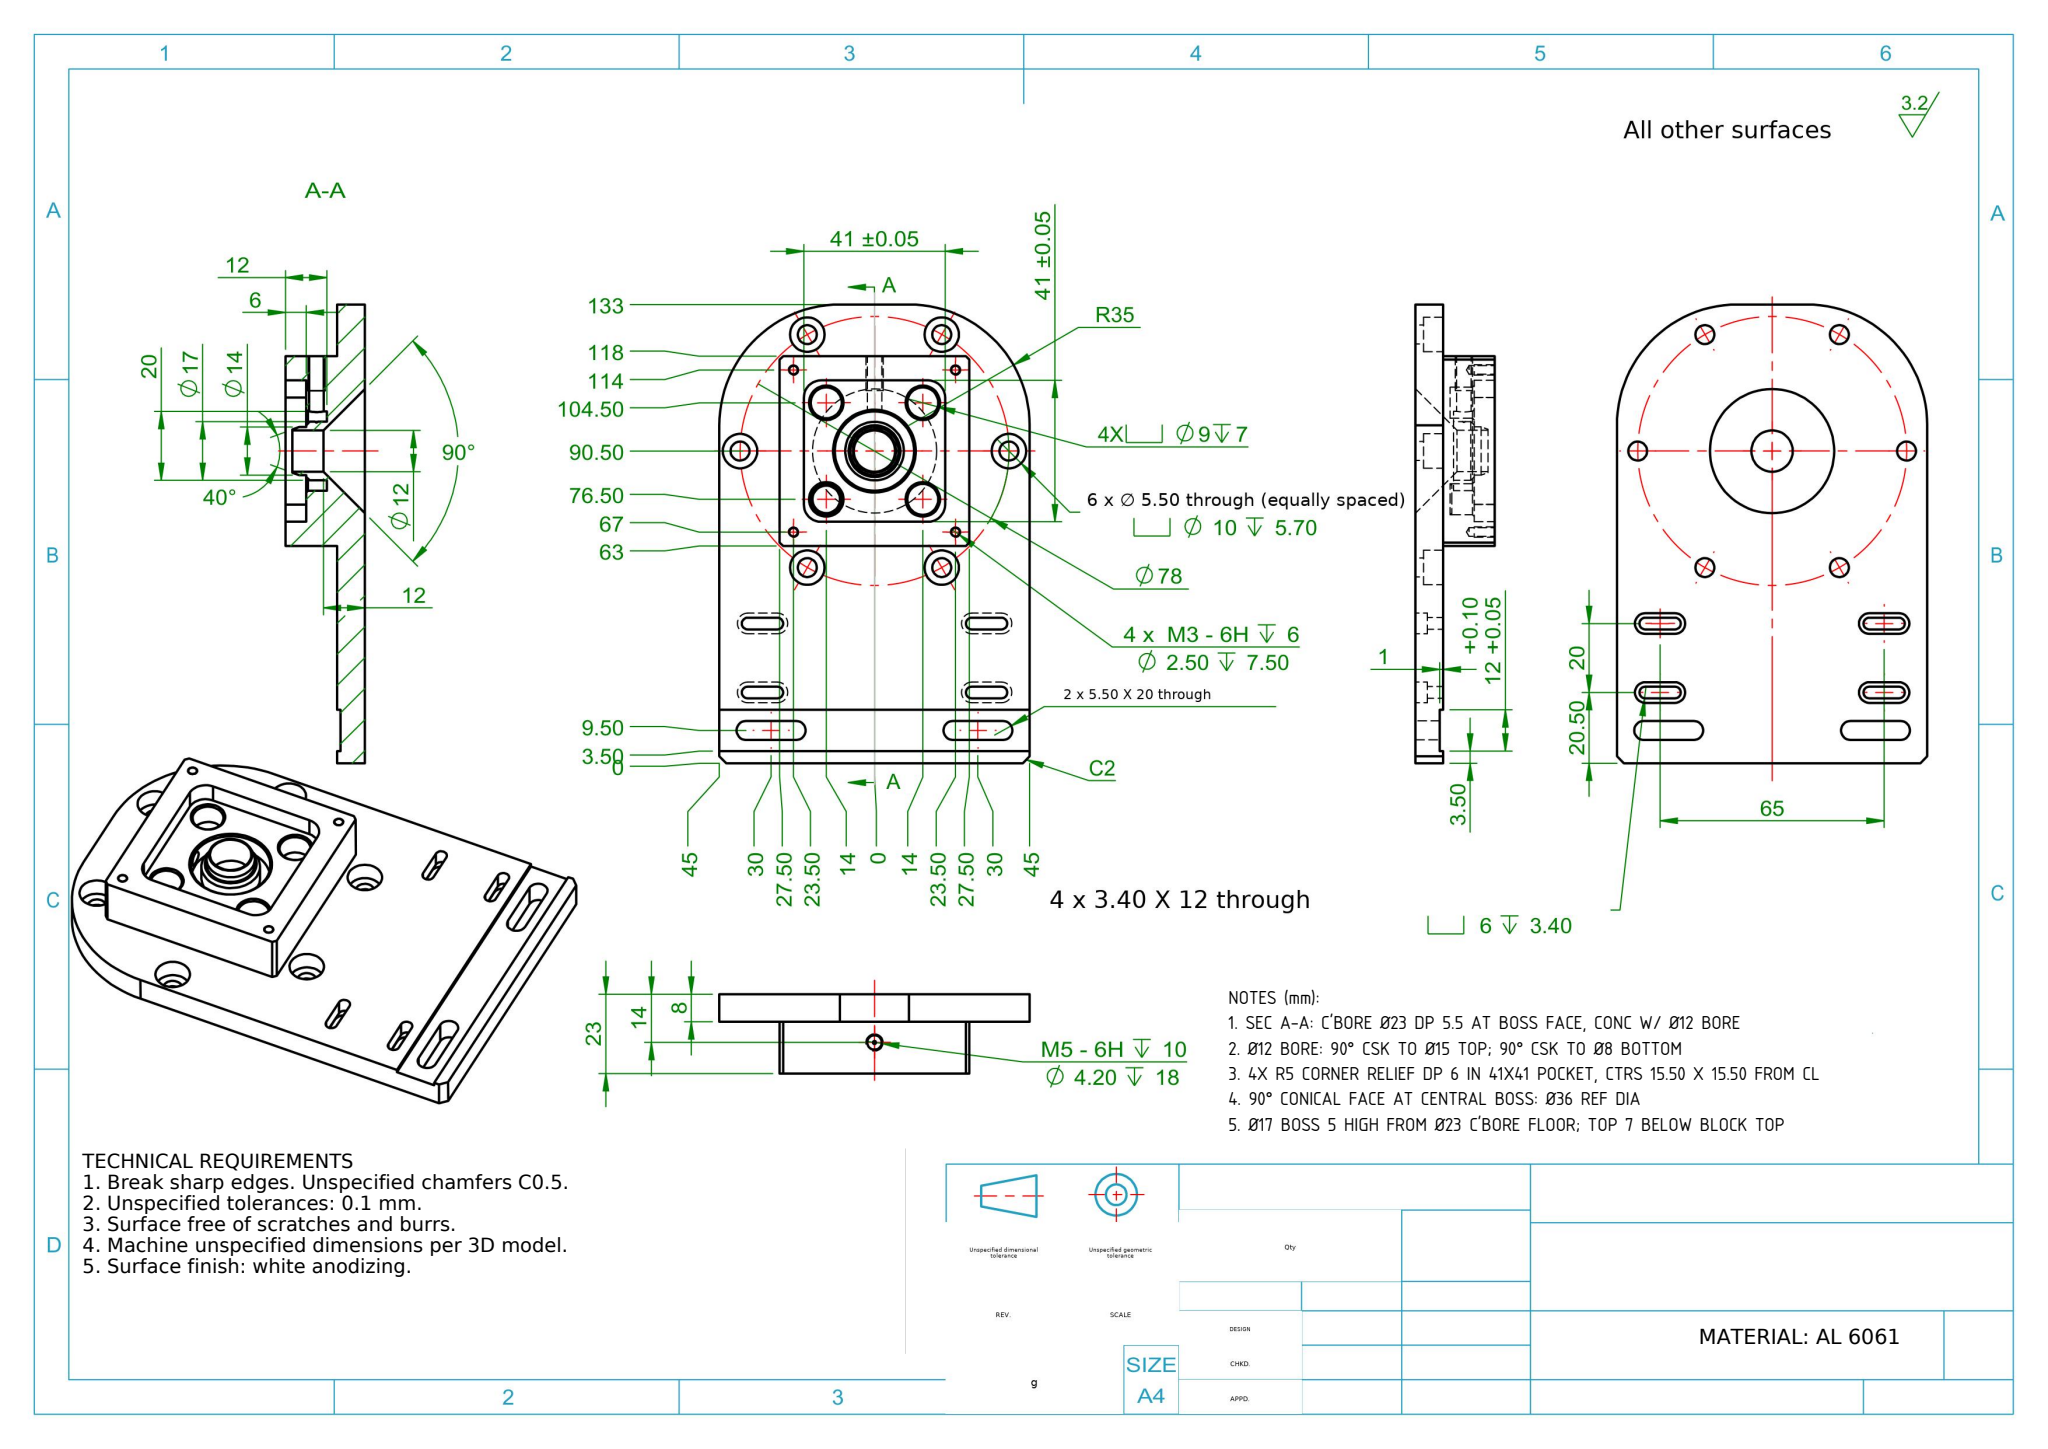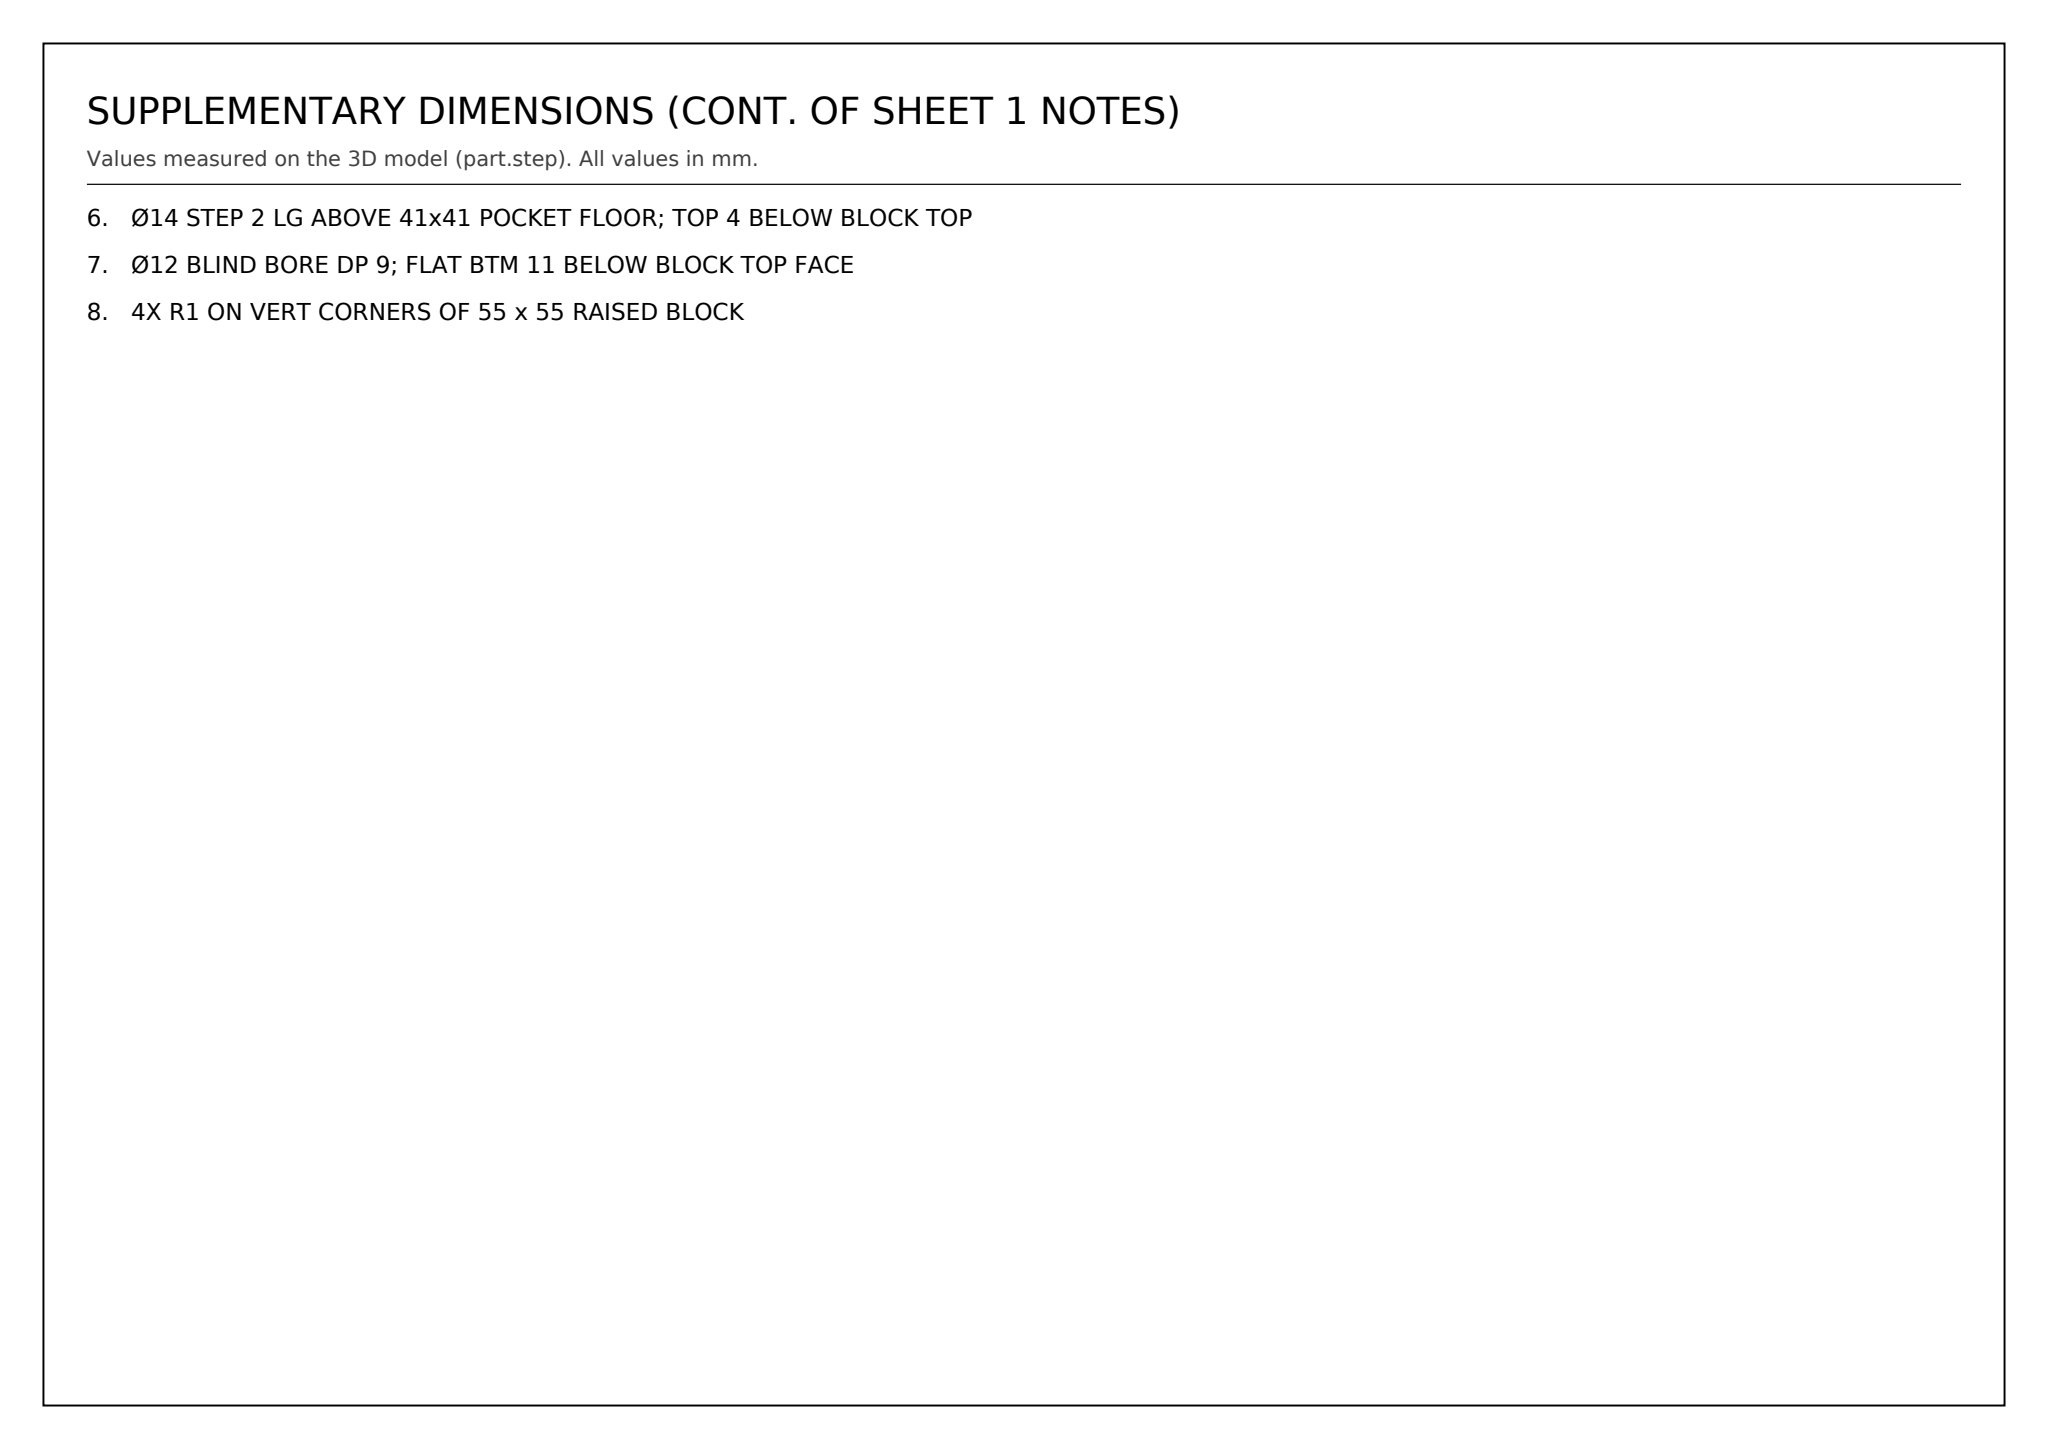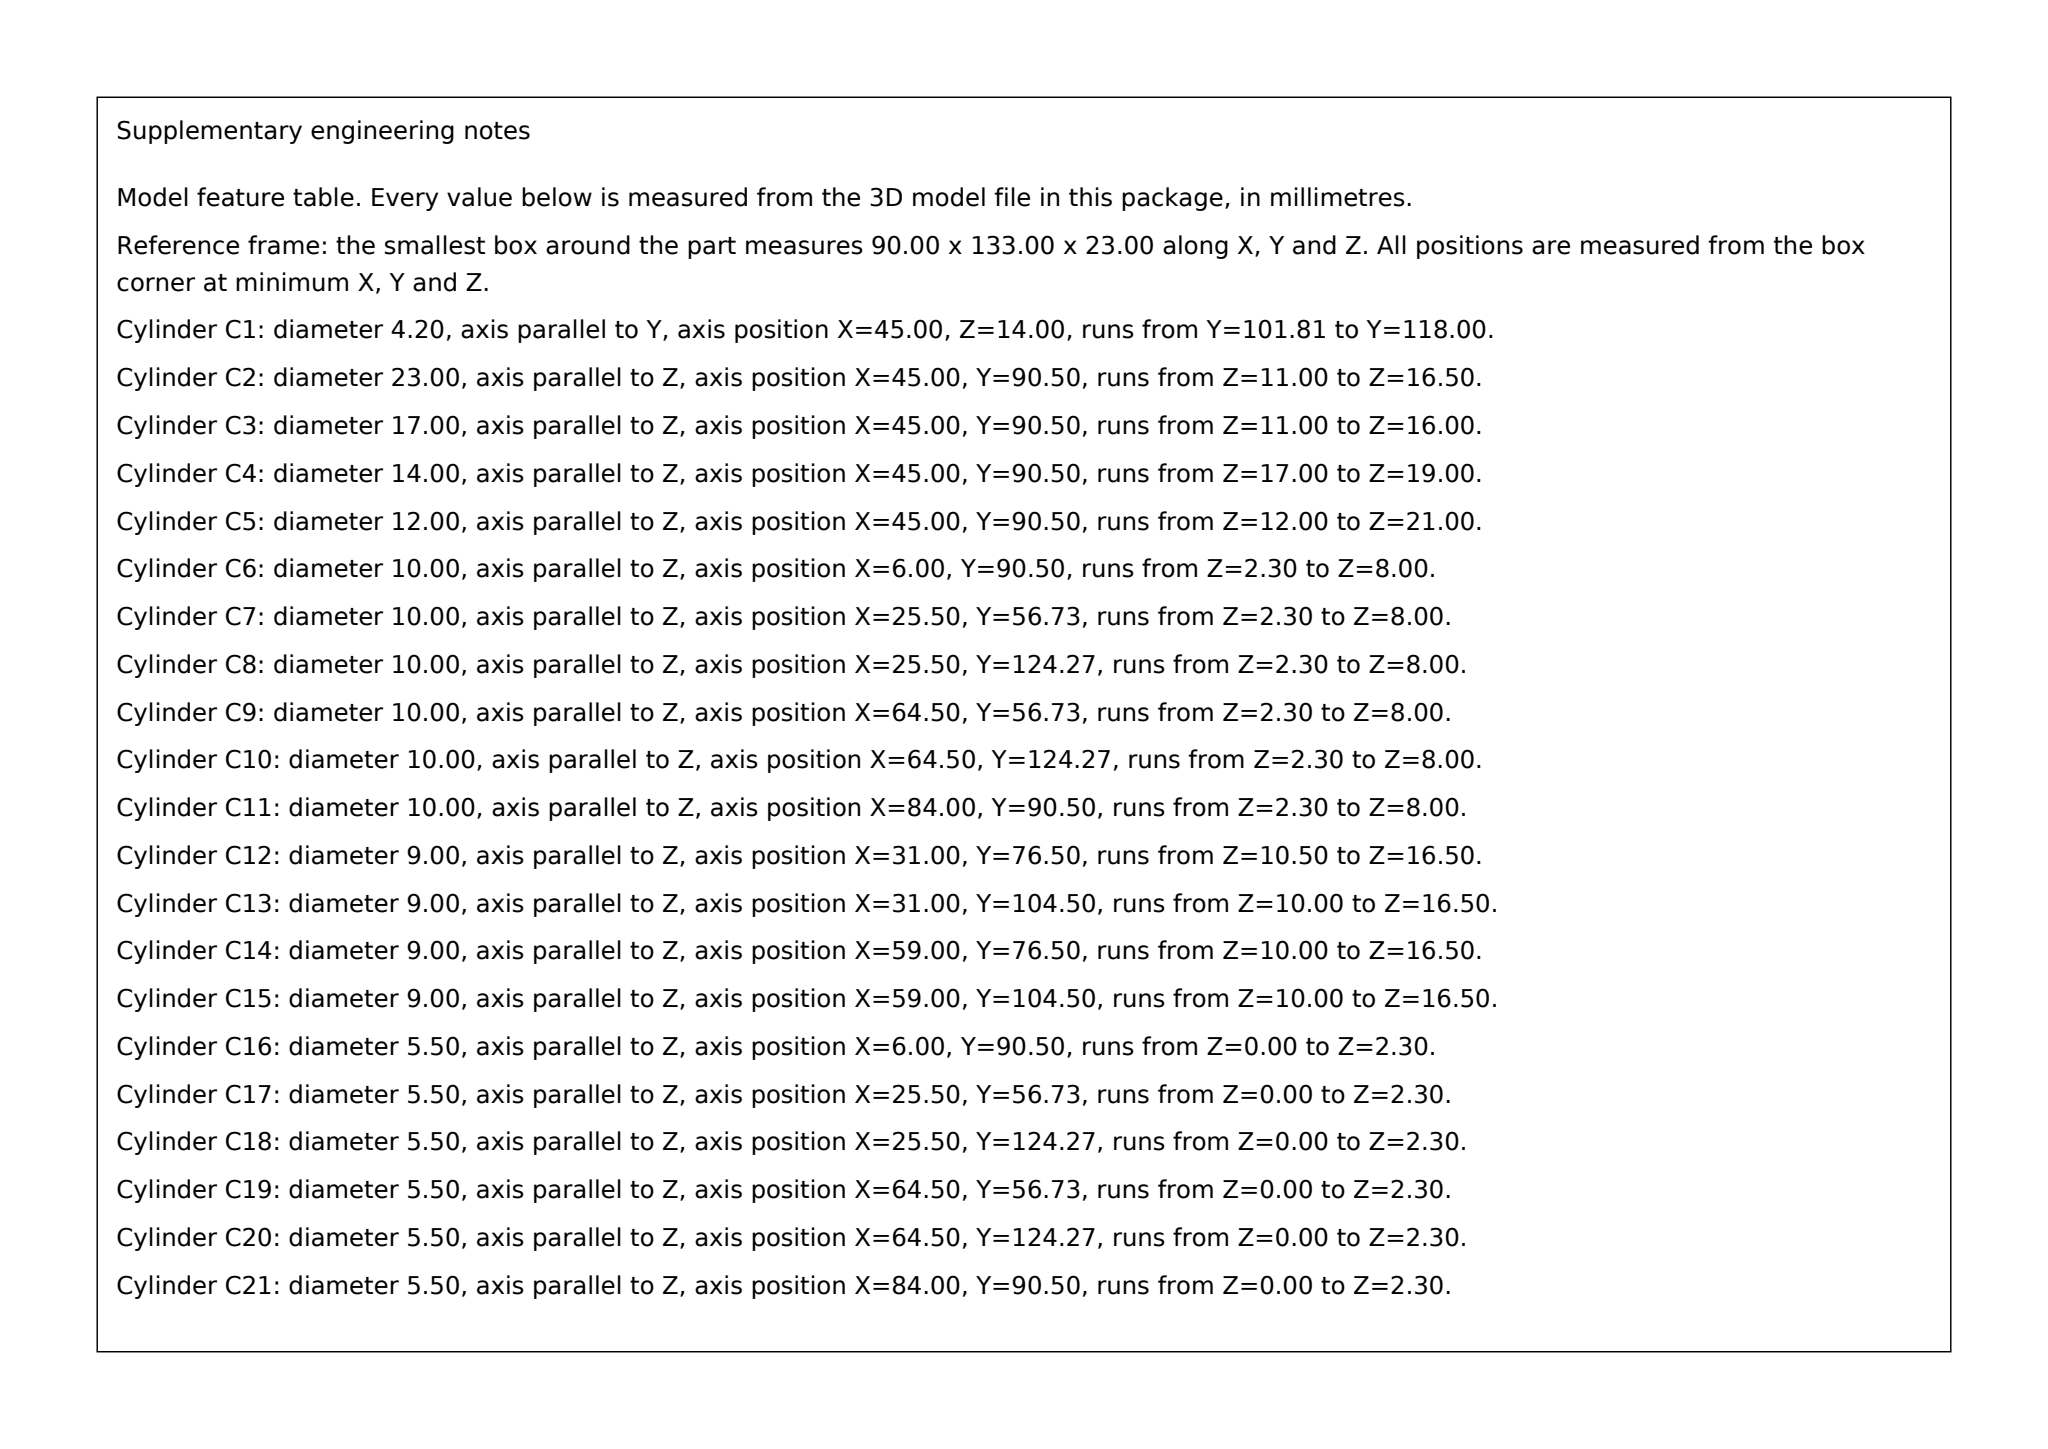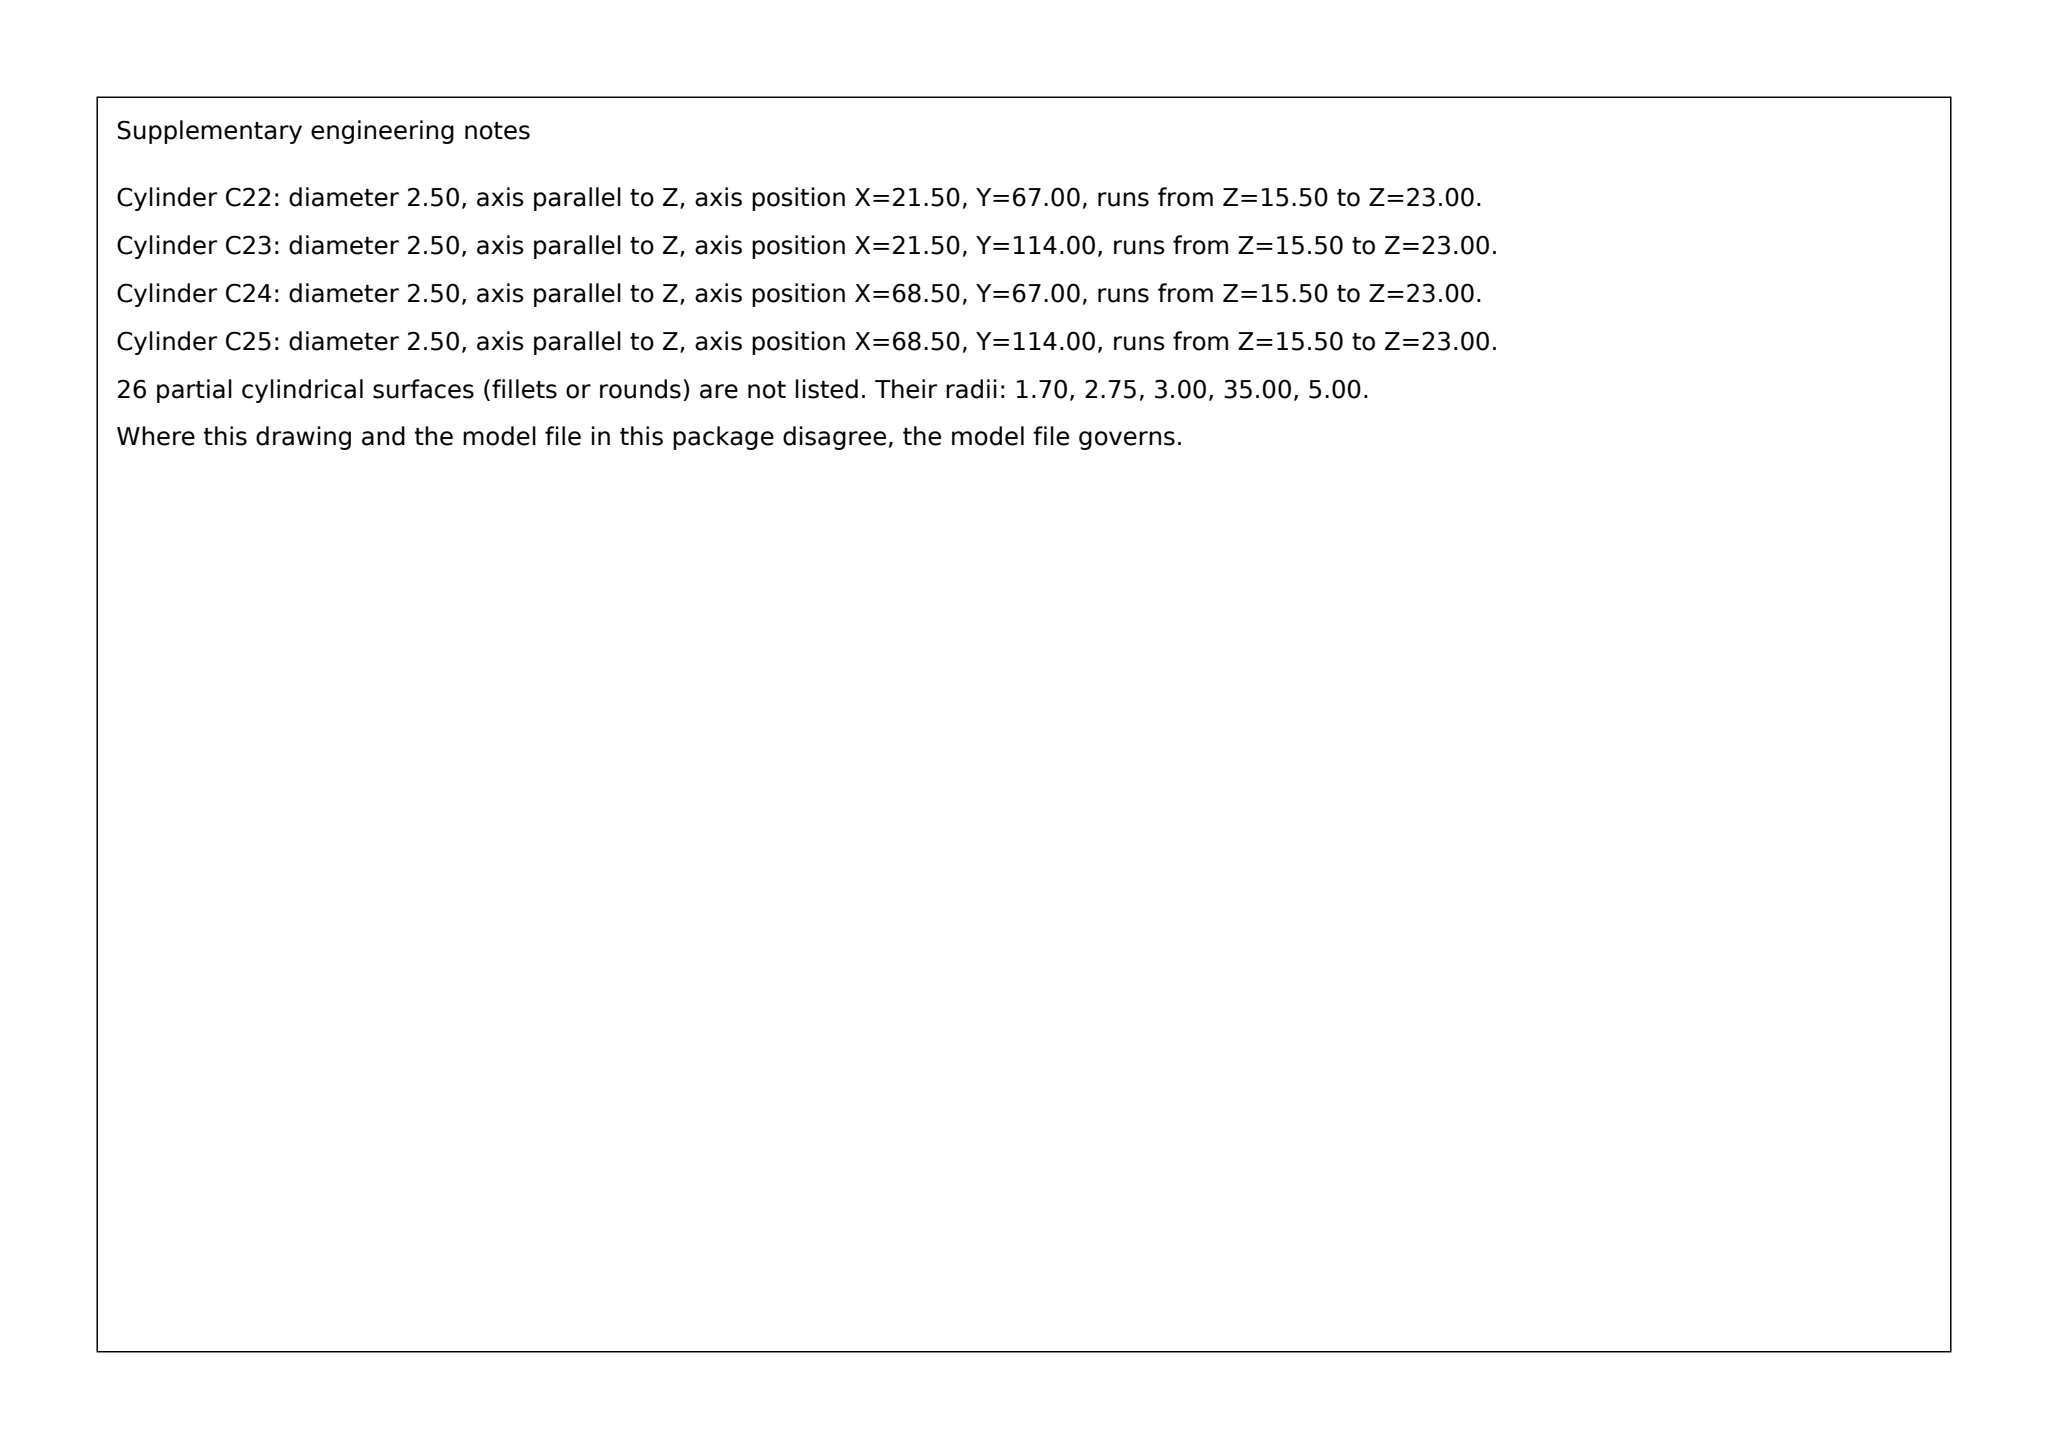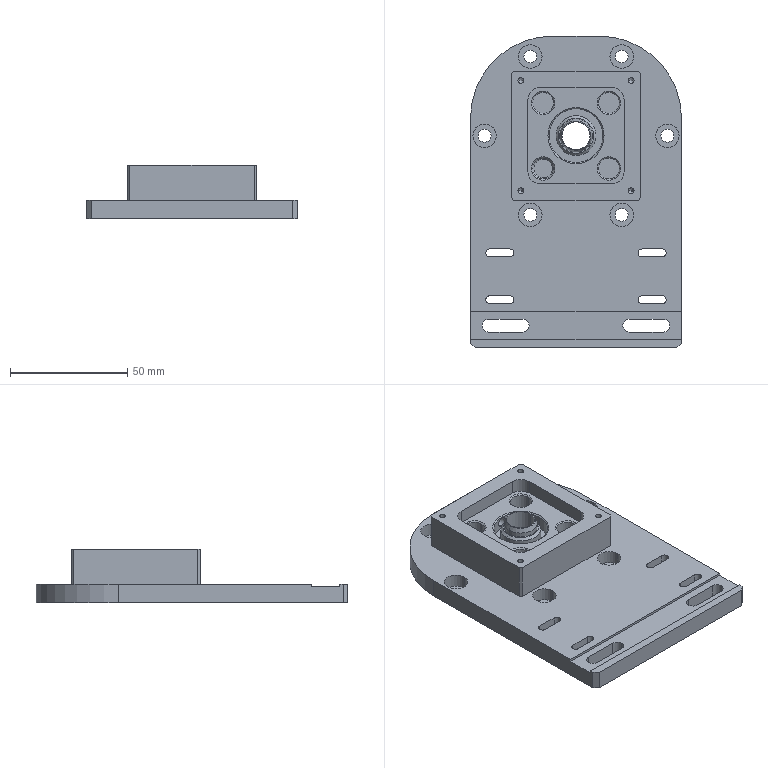Part | SolidWorks | mm | 1 solid | 177 faces | box 90 x 133 x 23 mm | volume 109928 mm3 | cylinder 86 | plane 63 | cone 28 | commonest cylinder face diameters 5.5 x18 10 x16 6 x12 3.4 x12 2.5 x8 9 x8 4.2 x2 17 x2
Drawing notes:
SEC A-A: C'BORE Ø23 DP 5.5 AT BOSS FACE, CONC W/ Ø12 BORE | from the solid: cylinder [23.0,"z",[45.0,90.5],5.5] coaxial with Ø17/Ø14/Ø12 bore at (45,90.5)
Ø12 BORE: 90° CSK TO Ø15 TOP; 90° CSK TO Ø8 BOTTOM | from the solid: cones [90.0,15.0] and [90.0,8.0] on Ø12 bore axis (45,90.5)
4X R5 CORNER RELIEF DP 6 IN 41X41 POCKET, CTRS 15.50 X 15.50 FROM CL | from the solid: Ø10 z-cylinders depth 6 at (29.5,75),(29.5,106),(60.5,75),(60.5,106); pocket 41x41 ctr (45,90.5), walls x=24.5/65.5, y=70/111
90° CONICAL FACE AT CENTRAL BOSS: Ø36 REF DIA | from the solid: cones[included_angle,ref_dia] entry [90.0, 36.0, 2] on central boss axis x=45, y=90.5
Ø17 BOSS 5 HIGH FROM Ø23 C'BORE FLOOR; TOP 7 BELOW BLOCK TOP | from the solid: cyl boss Ø17 z=11..16; bore Ø23 z=11..16.5 (floor z=11); block top plane z=23
Ø14 STEP 2 LG ABOVE 41x41 POCKET FLOOR; TOP 4 BELOW BLOCK TOP | from the solid: cyl Ø14 z=17..19; pocket floor plane z=17 (x24.5-65.5, y70-111); top face z=23
Ø12 BLIND BORE DP 9; FLAT BTM 11 BELOW BLOCK TOP FACE | from the solid: hole Ø12 z=12..21 (9 long, blind); top face plane z=23
4X R1 ON VERT CORNERS OF 55 x 55 RAISED BLOCK | from the solid: block x17.5-72.5 y63-118 z8-23; face x=17.5 extent y64-117, face y=118 extent x18.5-71.5 => 1 inset